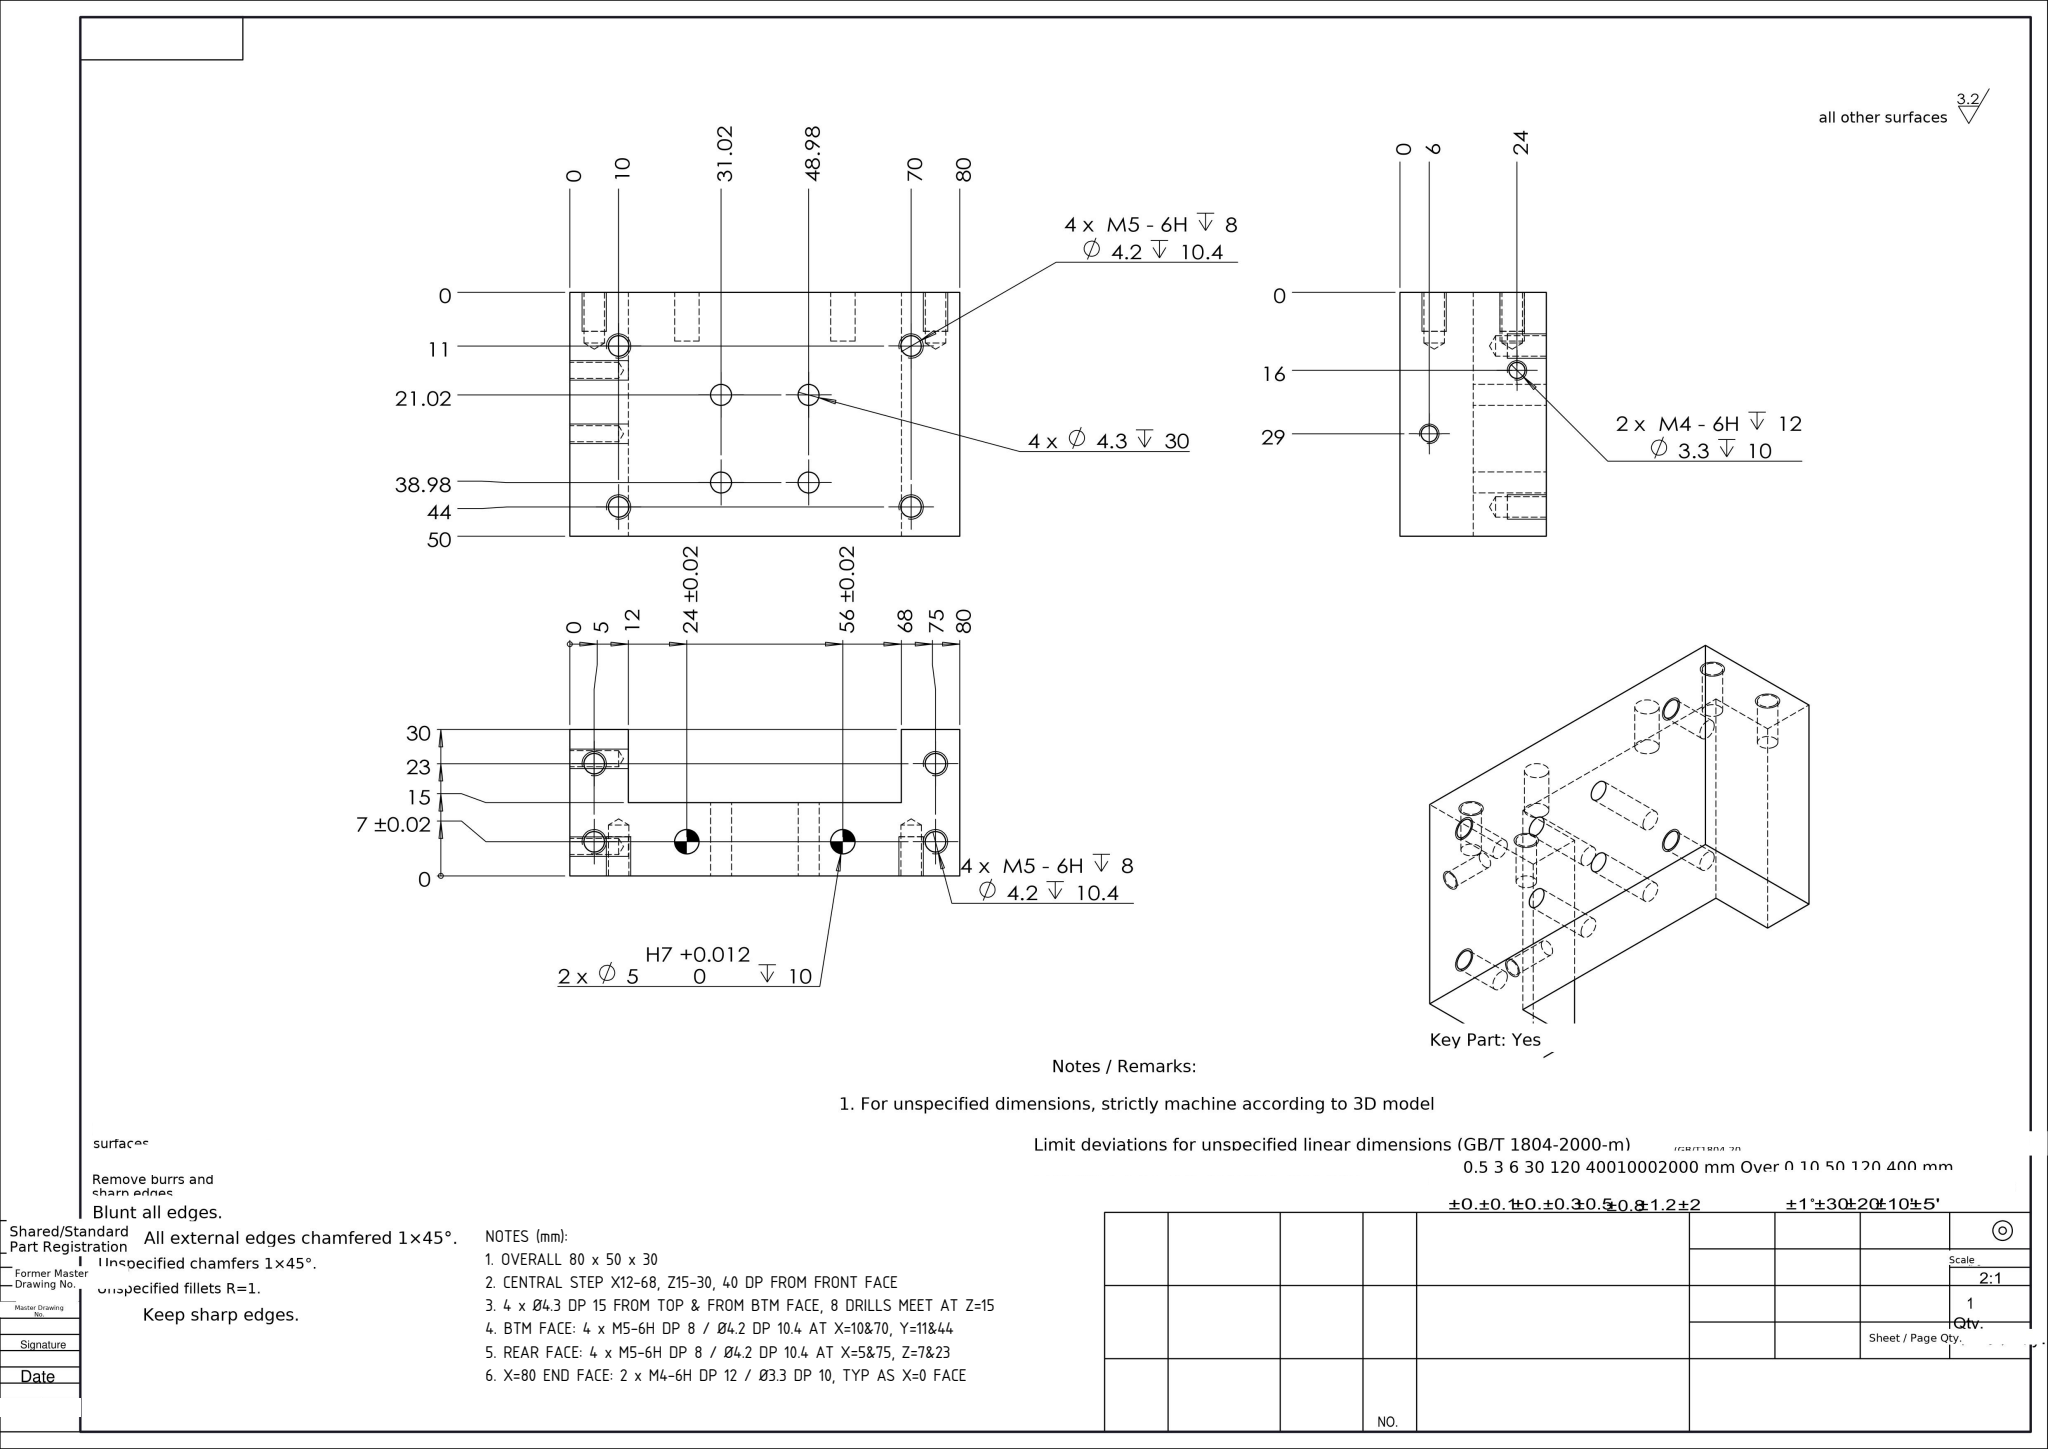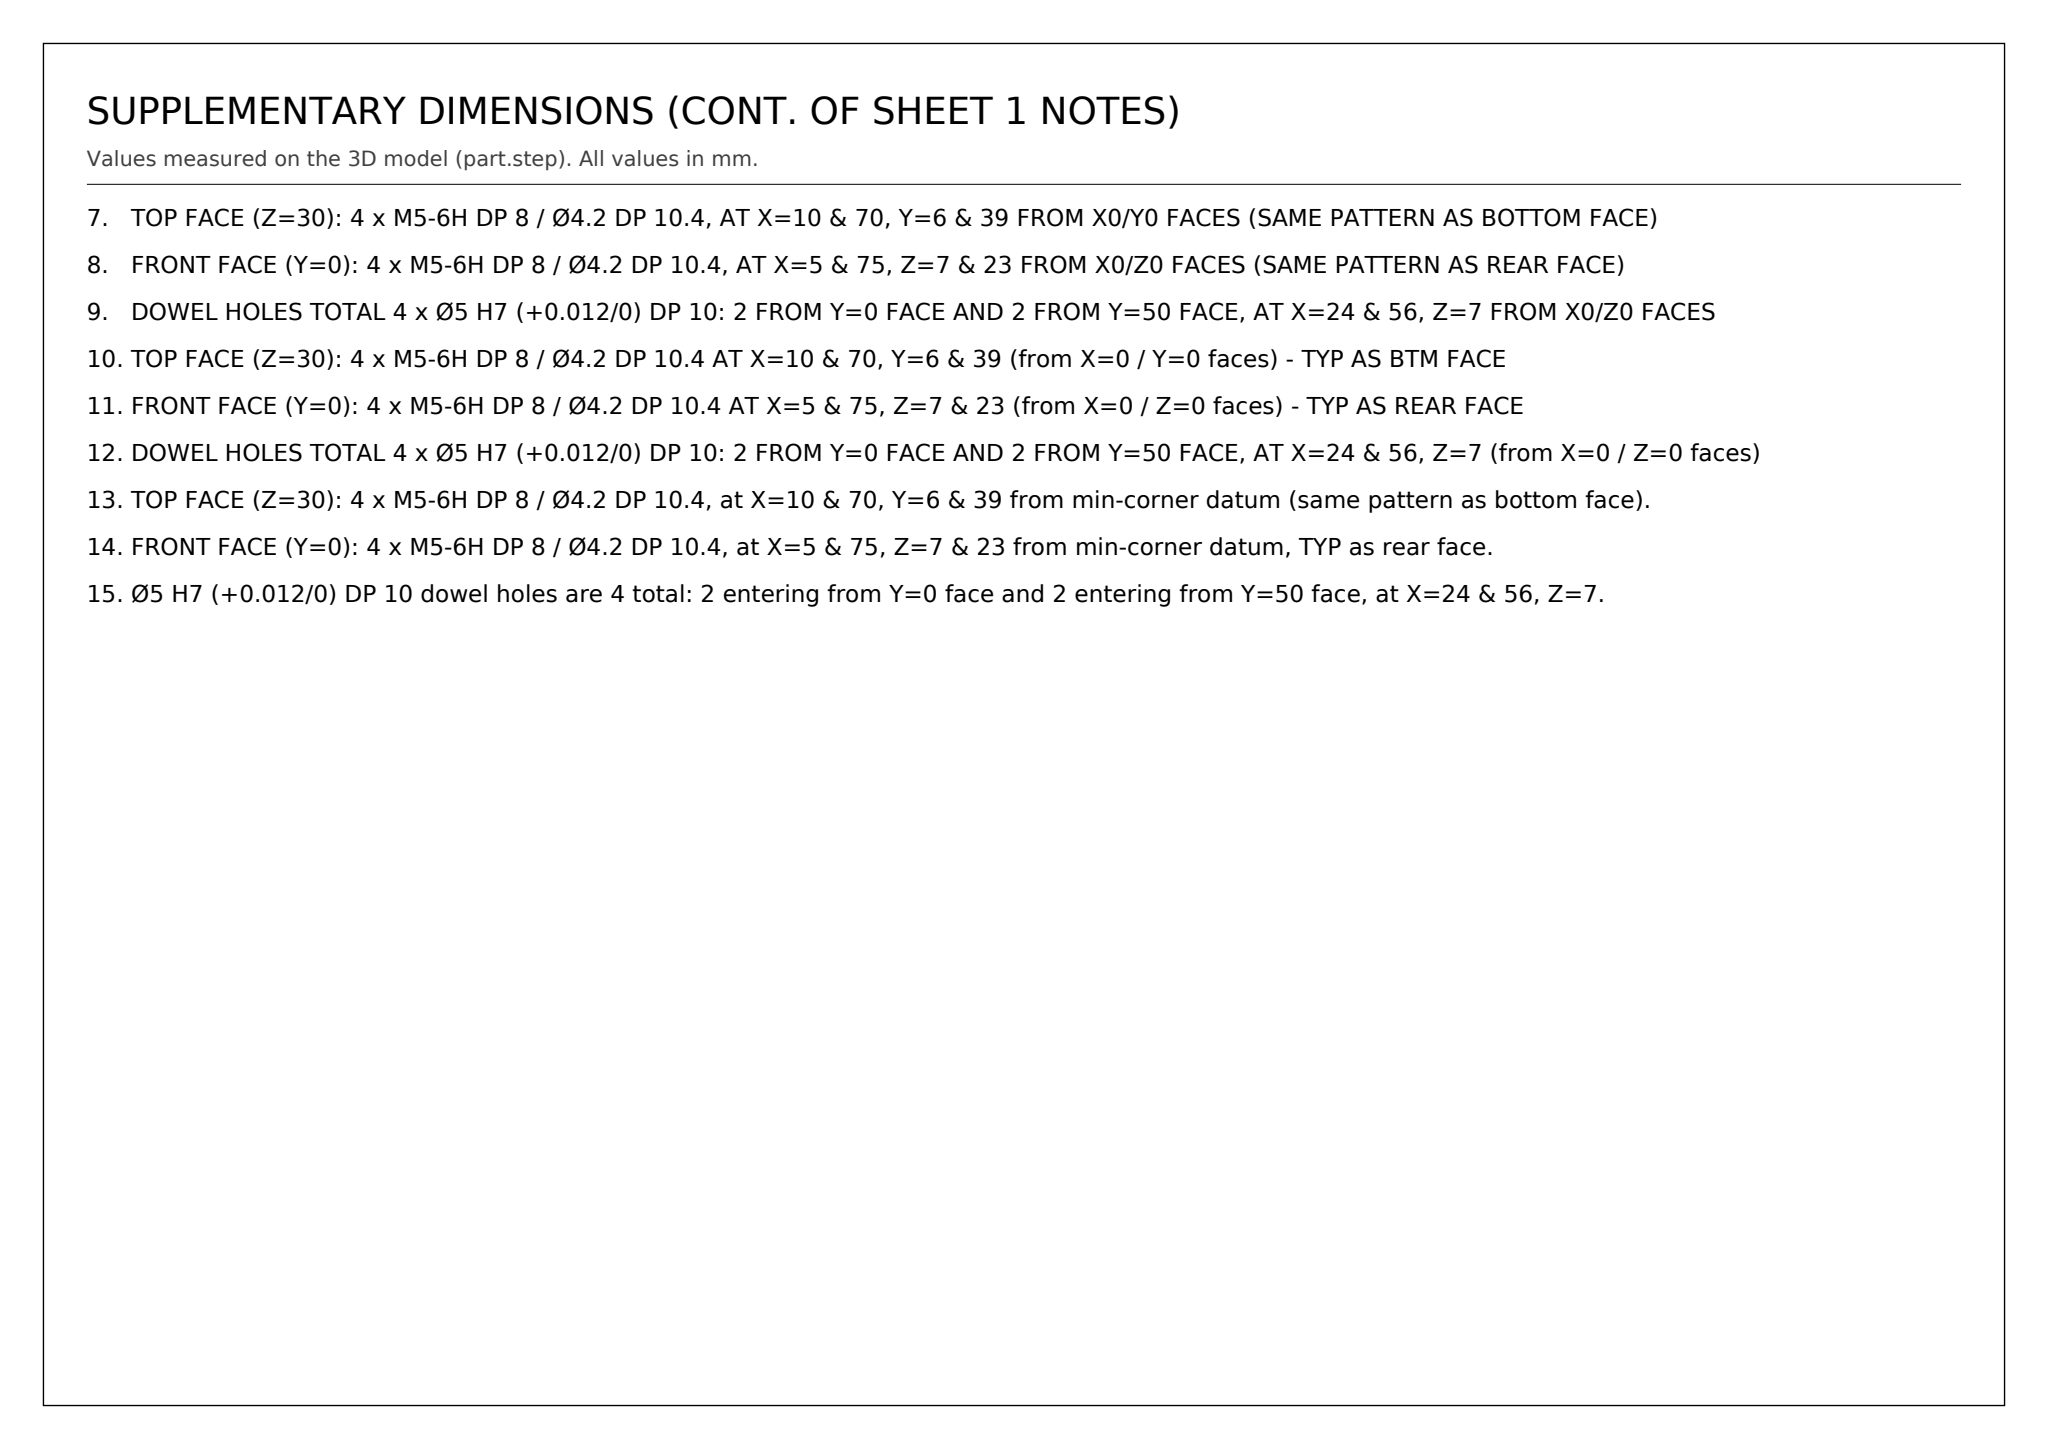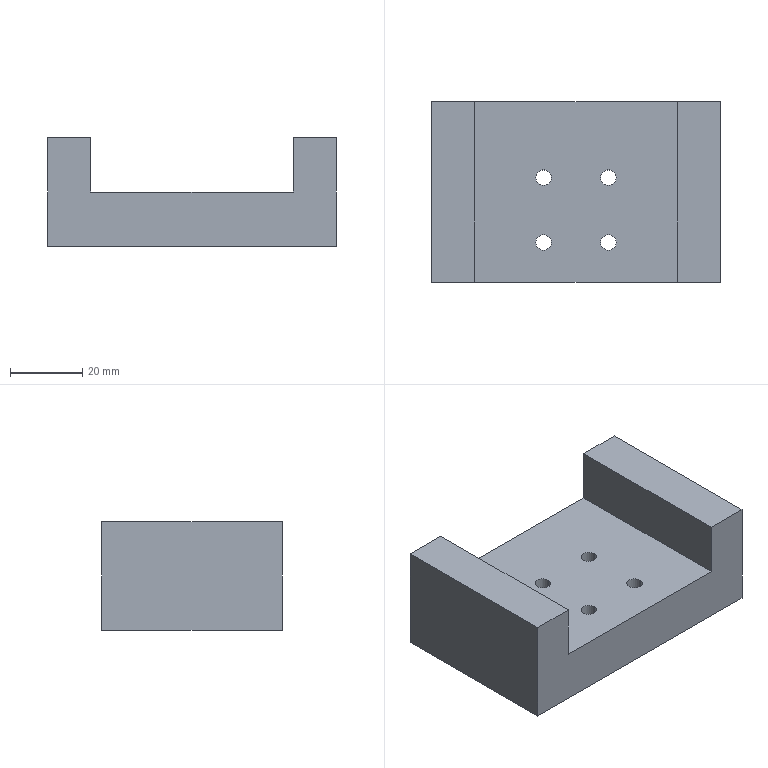Part | SolidWorks | mm | 1 solid | 64 faces | box 80 x 50 x 30 mm | volume 75360 mm3 | cylinder 32 | cone 20 | plane 12 | commonest cylinder face diameters 4.2 x16 4.3 x8 3.3 x4 5 x4
Drawing notes:
OVERALL 80 x 50 x 30 | from the solid: bbox_xyz [80,50,30]
CENTRAL STEP X12-68, Z15-30, 40 DP FROM FRONT FACE | from the solid: x planes 12 & 68, z planes 15 & 30, y planes 0/40 give 40 depth (back wall 40-50)
4 x Ø4.3 DP 15 FROM TOP & FROM BTM FACE, 8 DRILLS MEET AT Z=15 | from the solid: Ø4.3 z-axis cyls at (31.02,11.02),(31.02,28.98),(48.98,11.02),(48.98,28.98), L=15, count 2 each
BTM FACE: 4 x M5-6H DP 8 / Ø4.2 DP 10.4 AT X=10&70, Y=11&44 | from the solid: Ø4.2 z-axis cyls at (10,6),(10,39),(70,6),(70,39), L=10.4, count 2 each = 4 top + 4 btm
REAR FACE: 4 x M5-6H DP 8 / Ø4.2 DP 10.4 AT X=5&75, Z=7&23 | from the solid: Ø4.2 y-axis cyls at (5,7),(5,23),(75,7),(75,23), L=10.4, count 2 each = y=0 and y=50 faces
X=80 END FACE: 2 x M4-6H DP 12 / Ø3.3 DP 10, TYP AS X=0 FACE | from the solid: Ø3.3 x-axis cyls at (y21,z24),(y34,z6), L=10, count 2 each = both end faces x=0 and x=80
TOP FACE (Z=30): 4 x M5-6H DP 8 / Ø4.2 DP 10.4, AT X=10 & 70, Y=6 & 39 FROM X0/Y0 FACES (SAME PATTERN AS BOTTOM FACE) | from the solid: cylinders dia 4.2 axis z at [10,6],[10,39],[70,6],[70,39], length 10.4, count 2 each (one set per Z=0 and Z=30 face); cones 118° ref dia 4.2
FRONT FACE (Y=0): 4 x M5-6H DP 8 / Ø4.2 DP 10.4, AT X=5 & 75, Z=7 & 23 FROM X0/Z0 FACES (SAME PATTERN AS REAR FACE) | from the solid: cylinders dia 4.2 axis y at [5,7],[5,23],[75,7],[75,23], length 10.4, count 2 each (one set per Y=0 and Y=50 face)
DOWEL HOLES TOTAL 4 x Ø5 H7 (+0.012/0) DP 10: 2 FROM Y=0 FACE AND 2 FROM Y=50 FACE, AT X=24 & 56, Z=7 FROM X0/Z0 FACES | from the solid: cylinders dia 5.0 axis y at [24,7] and [56,7], length 10.0, count 2 each (entering from both Y faces)
TOP FACE (Z=30): 4 x M5-6H DP 8 / Ø4.2 DP 10.4 AT X=10 & 70, Y=6 & 39 (from X=0 / Y=0 faces) - TYP AS BTM FACE | from the solid: cylinders dia 4.2 axis z at [10,6],[10,39],[70,6],[70,39], length 10.4, count 2 each (one from Z=0, one from Z=30)
FRONT FACE (Y=0): 4 x M5-6H DP 8 / Ø4.2 DP 10.4 AT X=5 & 75, Z=7 & 23 (from X=0 / Z=0 faces) - TYP AS REAR FACE | from the solid: cylinders dia 4.2 axis y at [5,7],[5,23],[75,7],[75,23], length 10.4, count 2 each (one from Y=0, one from Y=50)
DOWEL HOLES TOTAL 4 x Ø5 H7 (+0.012/0) DP 10: 2 FROM Y=0 FACE AND 2 FROM Y=50 FACE, AT X=24 & 56, Z=7 (from X=0 / Z=0 faces) | from the solid: cylinders dia 5.0 axis y at [24,7] and [56,7], length 10.0, count 2 each
TOP FACE (Z=30): 4 x M5-6H DP 8 / Ø4.2 DP 10.4, at X=10 & 70, Y=6 & 39 from min-corner datum (same pattern as bottom face). | from the solid: cylinders dia 4.2 axis z at [10,6],[10,39],[70,6],[70,39], length 10.4, count 2 each (one set from Z=0, one from Z=30)
FRONT FACE (Y=0): 4 x M5-6H DP 8 / Ø4.2 DP 10.4, at X=5 & 75, Z=7 & 23 from min-corner datum, TYP as rear face. | from the solid: cylinders dia 4.2 axis y at [5,7],[5,23],[75,7],[75,23], length 10.4, count 2 each (one set from Y=0, one from Y=50)
Ø5 H7 (+0.012/0) DP 10 dowel holes are 4 total: 2 entering from Y=0 face and 2 entering from Y=50 face, at X=24 & 56, Z=7. | from the solid: cylinders dia 5.0 axis y at [24,7] and [56,7], length 10, count 2 each
build123d program:
from build123d import *

# Parameters (mm, degrees)
SKETCH1_W                     = 80
SKETCH1_H                     = 50
BOSS_EXTRUDE1_DEPTH           = 15
SKETCH4_W                     = 12
SKETCH4_H                     = 50
BOSS_EXTRUDE2_DEPTH           = 15
M4_CLEARANCE_HOLE1_D          = 4.3
M4_CLEARANCE_HOLE1_DEPTH      = 30
M5_TAPPED_HOLE1_D             = 4.2
M5_TAPPED_HOLE1_DEPTH         = 10.4
M5_TAPPED_HOLE1_TIP           = 1.262
M5_TAPPED_HOLE2_D             = 4.2
M5_TAPPED_HOLE2_DEPTH         = 10.4
M5_TAPPED_HOLE2_TIP           = 1.262
SIZE_MM_DOWEL_PIN_HOLE1_D     = 5
SIZE_MM_DOWEL_PIN_HOLE1_DEPTH = 10
M4_TAPPED_HOLE1_D             = 3.3
M4_TAPPED_HOLE1_DEPTH         = 10
M4_TAPPED_HOLE1_TIP           = 0.9914


with BuildPart() as part:
    # Sketch1 → Boss-Extrude1 (new body)
    with BuildSketch(Plane.XY):
        Rectangle(SKETCH1_W, SKETCH1_H)
    extrude(amount=BOSS_EXTRUDE1_DEPTH)

    # Sketch4 → Boss-Extrude2 (add)
    with BuildSketch(Plane.XY.offset(15)):
        with Locations((-34, 0)):
            Rectangle(SKETCH4_W, SKETCH4_H)
        with Locations((34, 0)):
            Rectangle(SKETCH4_W, SKETCH4_H)
    extrude(amount=BOSS_EXTRUDE2_DEPTH)

    # M4 Clearance Hole1
    with Locations(Plane.XY.offset(15)):
        with Locations((-8.98, 3.98), (8.98, 3.98), (-8.98, -13.98), (8.98, -13.98)):
            Hole(M4_CLEARANCE_HOLE1_D / 2, depth=M4_CLEARANCE_HOLE1_DEPTH)

    # M5 Tapped Hole1
    with Locations(Plane(origin=(0, 0, 0), x_dir=(-1, 0, 0), z_dir=(0, 0, -1))):
        with Locations((-30, 14), (-30, -19), (30, 14), (30, -19)):
            Hole(M5_TAPPED_HOLE1_D / 2, depth=M5_TAPPED_HOLE1_DEPTH)
            with Locations((0, 0, -(M5_TAPPED_HOLE1_DEPTH + M5_TAPPED_HOLE1_TIP / 2))):  # 118° drill point
                Cone(0, M5_TAPPED_HOLE1_D / 2, M5_TAPPED_HOLE1_TIP, mode=Mode.SUBTRACT)

    # M5 Tapped Hole2
    with Locations(Plane(origin=(0, 25, 0), x_dir=(1, 0, 0), z_dir=(0, 1, 0))):
        with Locations((-35, -7), (-35, -23), (35, -7), (35, -23)):
            Hole(M5_TAPPED_HOLE2_D / 2, depth=M5_TAPPED_HOLE2_DEPTH)
            with Locations((0, 0, -(M5_TAPPED_HOLE2_DEPTH + M5_TAPPED_HOLE2_TIP / 2))):  # 118° drill point
                Cone(0, M5_TAPPED_HOLE2_D / 2, M5_TAPPED_HOLE2_TIP, mode=Mode.SUBTRACT)

    # Size mm Dowel Pin Hole1
    with Locations(Plane(origin=(0, 25, 0), x_dir=(1, 0, 0), z_dir=(0, 1, 0))):
        with Locations((-16, -7), (16, -7)):
            Hole(SIZE_MM_DOWEL_PIN_HOLE1_D / 2, depth=SIZE_MM_DOWEL_PIN_HOLE1_DEPTH)

    # M4 Tapped Hole1
    with Locations(Plane(origin=(40, 0, 0), x_dir=(0, 0, -1), z_dir=(1, 0, 0))):
        with Locations((-6, 9), (-24, -4)):
            Hole(M4_TAPPED_HOLE1_D / 2, depth=M4_TAPPED_HOLE1_DEPTH)
            with Locations((0, 0, -(M4_TAPPED_HOLE1_DEPTH + M4_TAPPED_HOLE1_TIP / 2))):  # 118° drill point
                Cone(0, M4_TAPPED_HOLE1_D / 2, M4_TAPPED_HOLE1_TIP, mode=Mode.SUBTRACT)


solid = part.part